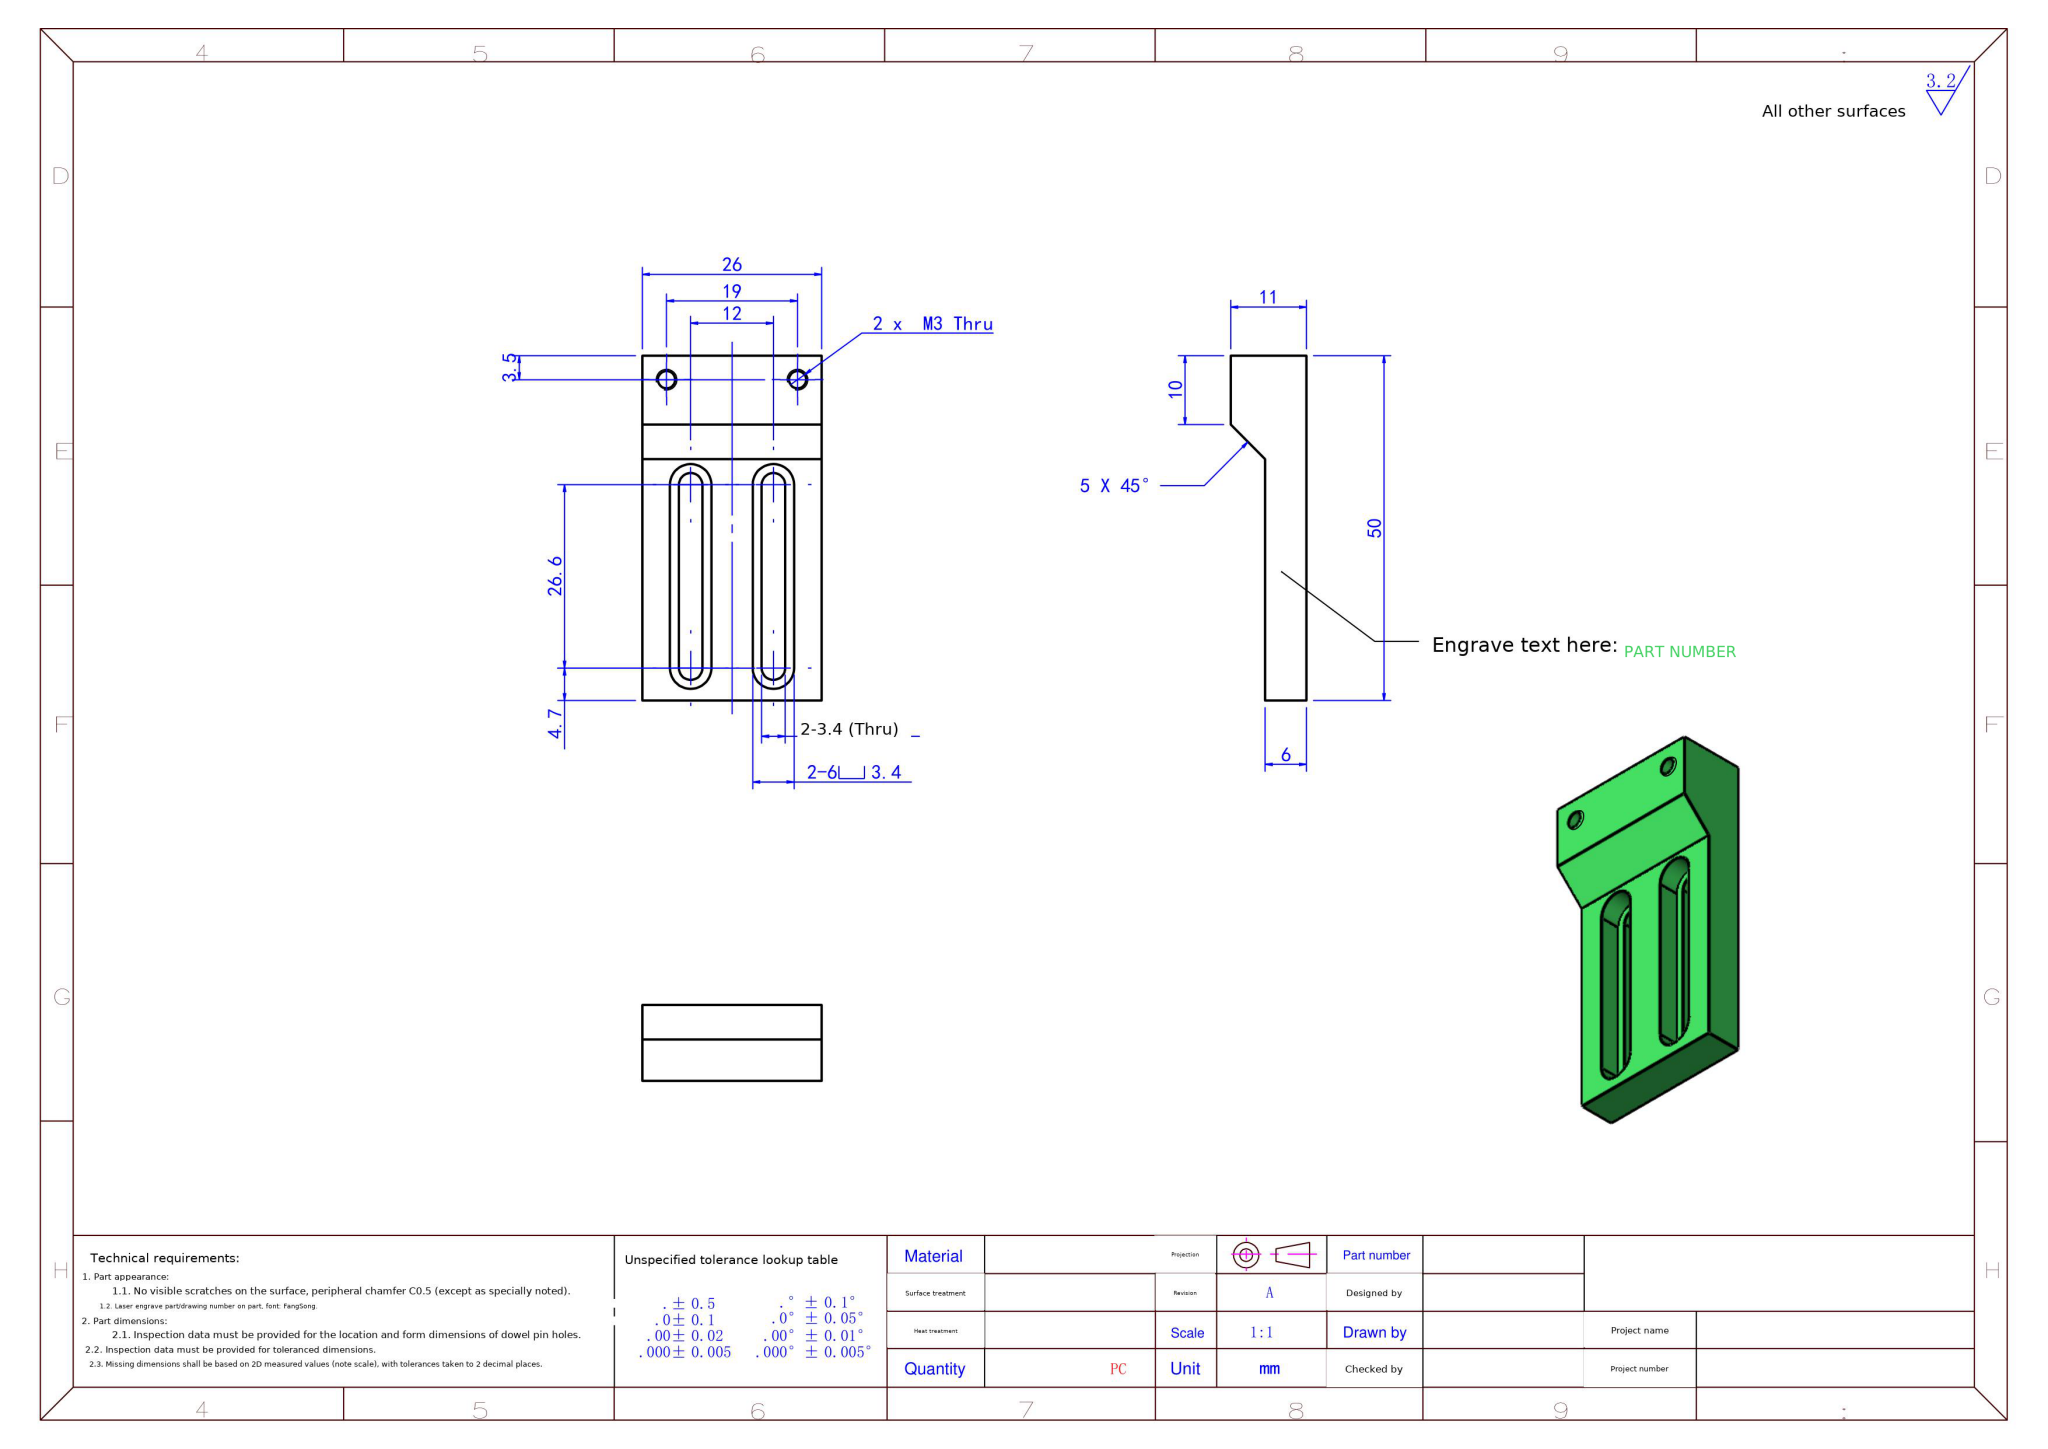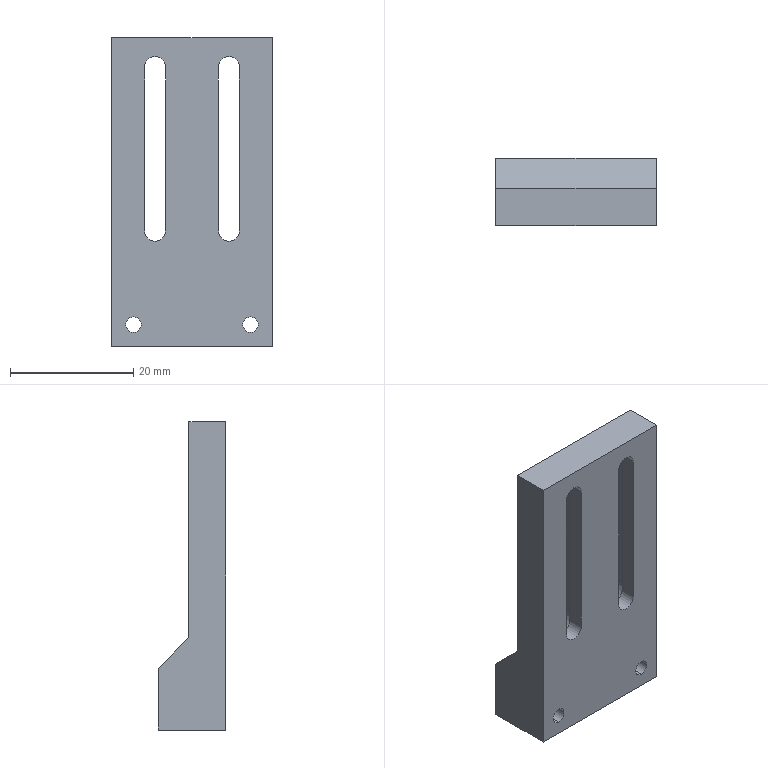Part | NX | mm | 1 solid | 34 faces | box 26 x 11 x 50 mm | volume 7522 mm3 | plane 18 | cylinder 16 | commonest cylinder face diameters 6 x6 3.4 x6 2.5 x4